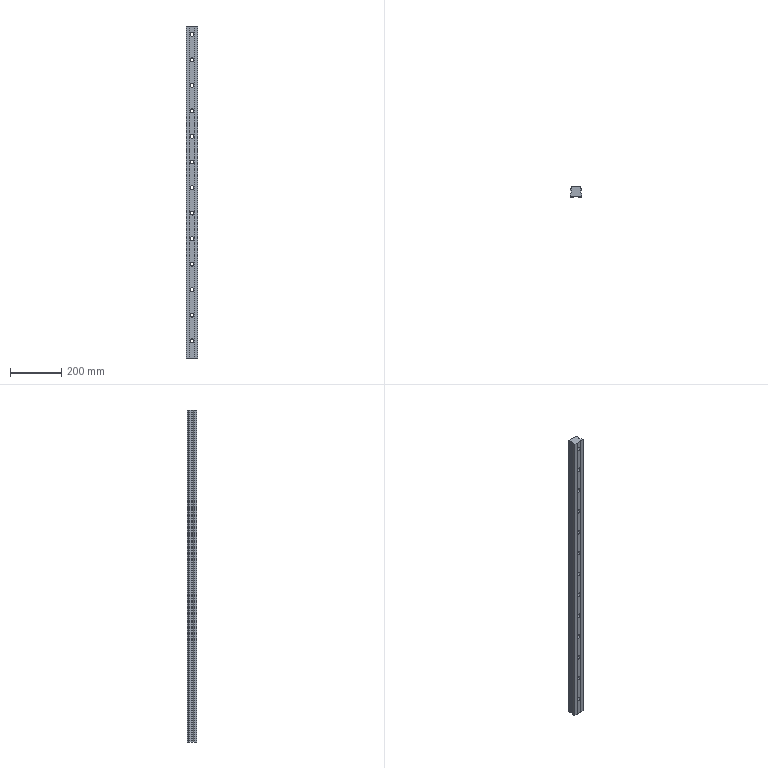Component | SolidWorks | GuideRail2100-1 | 1 solid | 86 faces | box 45 x 38 x 1300 mm | volume 1823830 mm3 | cylinder 55 | plane 31 | commonest cylinder face diameters 30 x26 15.5 x26 10 x3
build123d program:
from build123d import *

# Parameters (mm, degrees)
BOSS_EXTRUDE1_DEPTH                                  = 650
CYLINDRICAL_COUNTERSUNK_HOLE1_FOR_M18_HE_D           = 15.5
CYLINDRICAL_COUNTERSUNK_HOLE1_FOR_M18_HE_CBORE_D     = 30
CYLINDRICAL_COUNTERSUNK_HOLE1_FOR_M18_HE_CBORE_DEPTH = 10
LPATTERN1_COUNT                                      = 13
LPATTERN1_PITCH                                      = 100


with BuildPart() as part:
    # Sketch1 → Boss-Extrude1 (new, symmetric)
    with BuildSketch(Plane.XY):
        with BuildLine():
            Line((-10, -20.5), (10, -20.5))
            Line((10, -20.5), (10, -22))
            Line((10, -22), (22.5, -22))
            Line((22.5, -22), (22.5, -10.871))
            Line((22.5, -10.871), (17.629, -6))
            Line((17.629, -6), (17.629, 0))
            Line((17.629, 0), (22.5, 4.871))
            Line((22.5, 4.871), (22.5, 9.871))
            ThreePointArc((22.5, 9.871), (18.586, 11.76), (17.629, 16))
            Line((17.629, 16), (-17.629, 16))
            ThreePointArc((-17.629, 16), (-18.586, 11.76), (-22.5, 9.871))
            Line((-22.5, 9.871), (-22.5, 4.871))
            Line((-22.5, 4.871), (-17.629, 0))
            Line((-17.629, 0), (-17.629, -6))
            Line((-17.629, -6), (-22.5, -10.871))
            Line((-22.5, -10.871), (-22.5, -22))
            Line((-22.5, -22), (-10, -22))
            Line((-10, -22), (-10, -20.5))
        make_face()
    extrude(amount=BOSS_EXTRUDE1_DEPTH, both=True)

    # Cylindrical Countersunk Hole1 for M18 He (through all)
    with Locations(Plane(origin=(0, 16, 0), x_dir=(-1, 0, 0), z_dir=(0, 1, 0))):
        with Locations((0, 617.5)):
            cylindrical_countersunk_hole1_for_m18_he = CounterBoreHole(CYLINDRICAL_COUNTERSUNK_HOLE1_FOR_M18_HE_D / 2, CYLINDRICAL_COUNTERSUNK_HOLE1_FOR_M18_HE_CBORE_D / 2, CYLINDRICAL_COUNTERSUNK_HOLE1_FOR_M18_HE_CBORE_DEPTH)

    # LPattern1: Cylindrical Countersunk Hole1 for M18 He ×13
    with Locations(*[(0, 0, -i * LPATTERN1_PITCH) for i in range(1, LPATTERN1_COUNT)]):
        add(cylindrical_countersunk_hole1_for_m18_he, mode=Mode.SUBTRACT)


solid = part.part

# Placed as in the assembly
solid = solid.moved(Location((-23.706, -230.275, 1030), (0, 0, 0)))